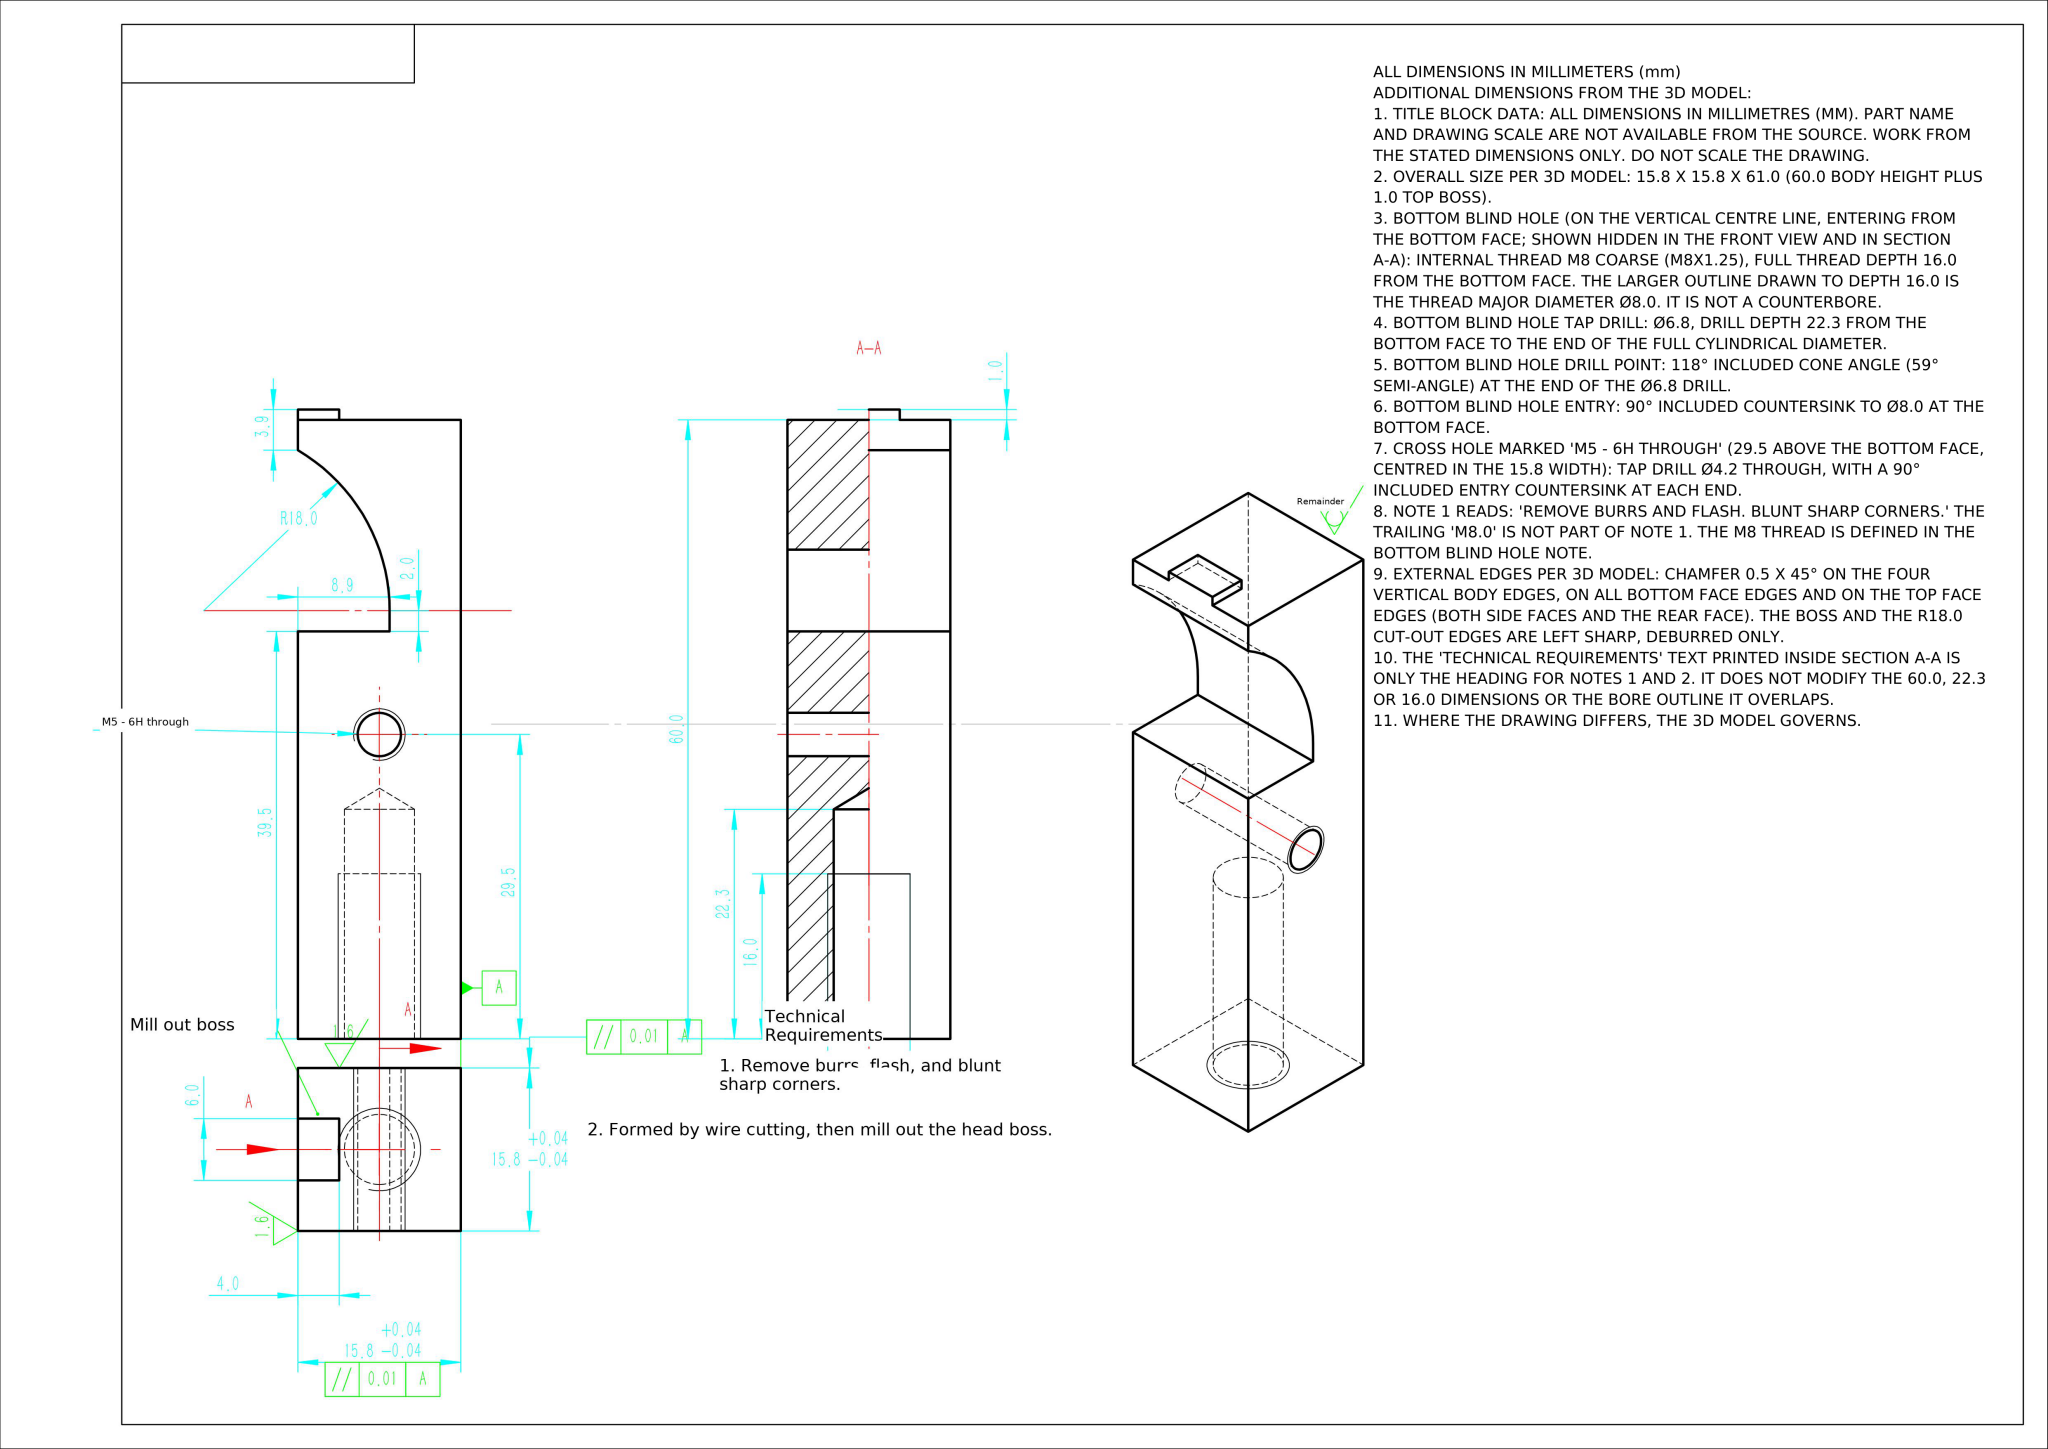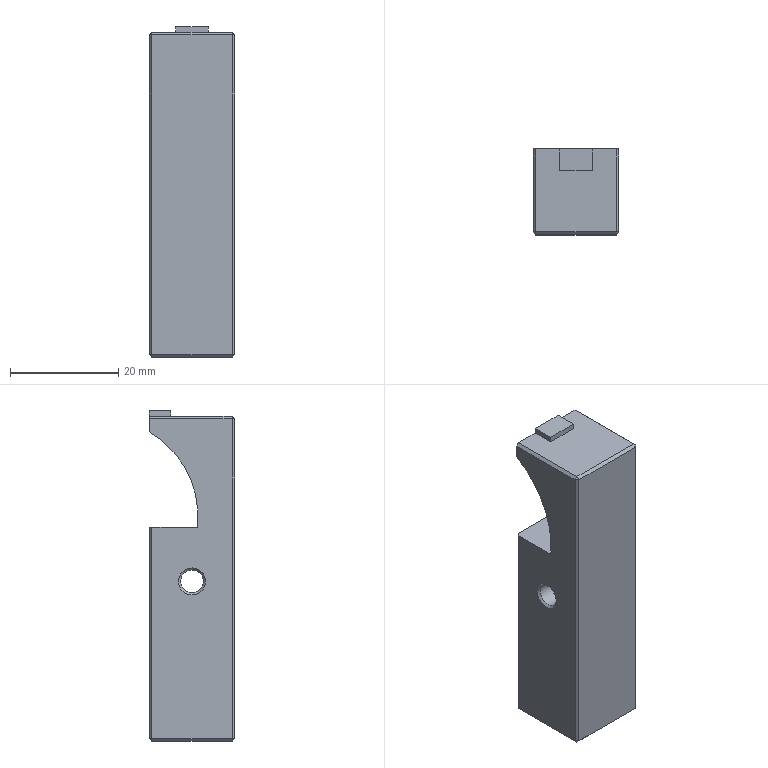Part | NX | mm | Stepped Tapered Tower Housing | 1 solid | 36 faces | box 15.8 x 15.8 x 61 mm | volume 12046 mm3 | plane 29 | cone 4 | cylinder 3 | commonest cylinder face diameters 36 x1 4.2 x1 6.8 x1